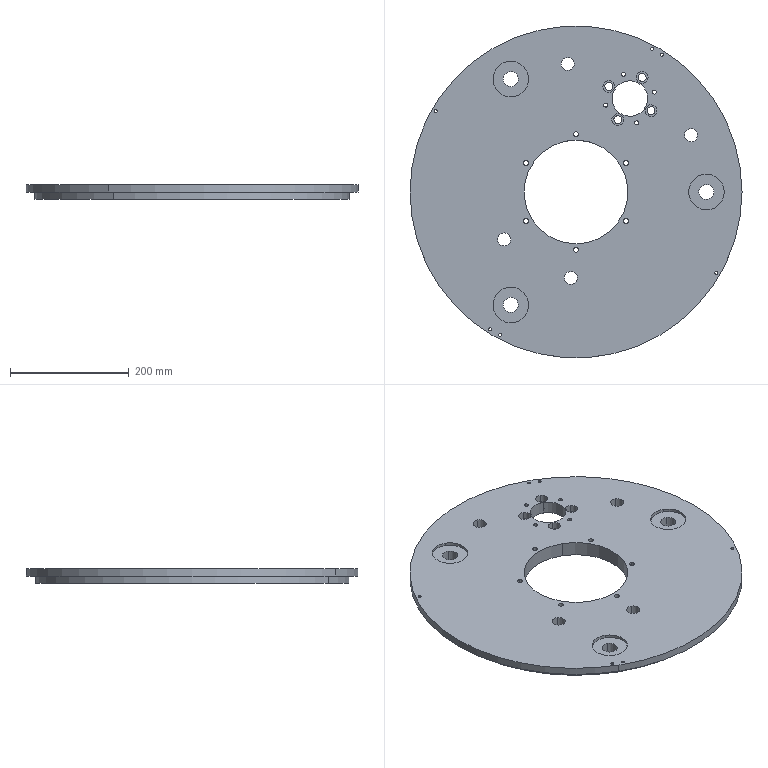Component | SolidWorks | KLHFH002Turntable-1 | 1 solid | 89 faces | box 560 x 560 x 25 mm | volume 4987410 mm3 | cylinder 78 | plane 11 | commonest cylinder face diameters 8.5 x12 5 x12 22 x8 60 x8 20 x8 6.8 x8 13.5 x8 25.5 x6 | material Plain Carbon Steel
build123d program:
from build123d import *

# Parameters (mm, degrees)
SKETCH1_R                                          = 265
BOSS_EXTRUDE1_DEPTH                                = 12.5
SKETCH2_R                                          = 30
SKETCH2_R_2                                        = 35
CUT_EXTRUDE1_DEPTH                                 = 376.6
HOLE_SIZE_ACCORDING_TO_TYPE_1_OF_HEXAG_D           = 13.5
HOLE_SIZE_ACCORDING_TO_TYPE_1_OF_HEXAG_DEPTH       = 38.75
HOLE_SIZE_ACCORDING_TO_TYPE_1_OF_HEXAG_CBORE_D     = 20
HOLE_SIZE_ACCORDING_TO_TYPE_1_OF_HEXAG_CBORE_DEPTH = 13
HOLE_SIZE_ACCORDING_TO_TYPE_1_OF_HEXAG_TIP         = 4.056
M8_TAPPED_HOLE1_D                                  = 6.8
SKETCH7_R                                          = 65
CUT_EXTRUDE2_DEPTH                                 = 3
HOLE_SIZE_ACCORDING_TO_TYPE_2_OF_HEXAG_D           = 9
HOLE_SIZE_ACCORDING_TO_TYPE_2_OF_HEXAG_CBORE_D     = 15
HOLE_SIZE_ACCORDING_TO_TYPE_2_OF_HEXAG_CBORE_DEPTH = 9
SKETCH10_R                                         = 8
CUT_EXTRUDE3_DEPTH                                 = 3
M6_TAPPED_HOLE2_D                                  = 5
SKETCH15_R                                         = 30
CUT_EXTRUDE4_DEPTH                                 = 5
F_25_5_25_5_DIAMETER_HOLE1_D                       = 25.5
CIRPATTERN1_COUNT                                  = 3
M10_TAPPED_HOLE1_D                                 = 8.5
SKETCH20_R                                         = 11
CUT_EXTRUDE5_DEPTH                                 = 376.6
SKETCH21_R                                         = 11
CUT_EXTRUDE6_DEPTH                                 = 376.6
BOSS_EXTRUDE2_START                                = -12.5
SKETCH22_R                                         = 280
SKETCH22_R_2                                       = 265
BOSS_EXTRUDE2_DEPTH                                = 12.5
M6_TAPPED_HOLE3_D                                  = 5
SKETCH25_R                                         = 87.5
CUT_EXTRUDE7_DEPTH                                 = 397.768
M10_TAPPED_HOLE2_D                                 = 8.5
CIRPATTERN2_COUNT                                  = 6


with BuildPart() as part:
    # Sketch1 → Boss-Extrude1 (new, symmetric)
    with BuildSketch(Plane.XY):
        Circle(SKETCH1_R)
    extrude(amount=BOSS_EXTRUDE1_DEPTH, both=True)

    # Sketch2 → Cut-Extrude1 (cut, through all)
    with BuildSketch(Plane.XY.offset(12.5)):
        with Locations((-182, 0)):
            Circle(SKETCH2_R)
        Circle(SKETCH2_R_2)
    extrude(amount=-CUT_EXTRUDE1_DEPTH, mode=Mode.SUBTRACT)

    # Hole Size _according to_ Type 1 of Hexag
    with Locations(Plane(origin=(0, 0, -12.5), x_dir=(-1, 0, 0), z_dir=(0, 0, -1))):
        with Locations((141, 0), (182, 41), (223, 0), (182, -41)):
            CounterBoreHole(HOLE_SIZE_ACCORDING_TO_TYPE_1_OF_HEXAG_D / 2, HOLE_SIZE_ACCORDING_TO_TYPE_1_OF_HEXAG_CBORE_D / 2, HOLE_SIZE_ACCORDING_TO_TYPE_1_OF_HEXAG_CBORE_DEPTH, depth=HOLE_SIZE_ACCORDING_TO_TYPE_1_OF_HEXAG_DEPTH)
            with Locations((0, 0, -(HOLE_SIZE_ACCORDING_TO_TYPE_1_OF_HEXAG_DEPTH + HOLE_SIZE_ACCORDING_TO_TYPE_1_OF_HEXAG_TIP / 2))):  # 118° drill point
                Cone(0, HOLE_SIZE_ACCORDING_TO_TYPE_1_OF_HEXAG_D / 2, HOLE_SIZE_ACCORDING_TO_TYPE_1_OF_HEXAG_TIP, mode=Mode.SUBTRACT)

    # M8 Tapped Hole1 (through all)
    with Locations(Plane(origin=(0, 0, -12.5), x_dir=(-1, 0, 0), z_dir=(0, 0, -1))):
        with Locations((212, 30), (212, -30), (152, -30), (152, 30)):
            Hole(M8_TAPPED_HOLE1_D / 2)

    # Sketch7 → Cut-Extrude2 (cut)
    with BuildSketch(Plane.XY.offset(12.5)):
        with Locations((-182, 0)):
            Circle(SKETCH7_R)
    extrude(amount=-CUT_EXTRUDE2_DEPTH, mode=Mode.SUBTRACT)

    # Hole Size _according to_ Type 2 of Hexag (through all)
    with Locations(Plane(origin=(0, 0, -12.5), x_dir=(1, 0, 0), z_dir=(0, 0, -1))):
        with Locations((-50, 0), (50, 0)):
            CounterBoreHole(HOLE_SIZE_ACCORDING_TO_TYPE_2_OF_HEXAG_D / 2, HOLE_SIZE_ACCORDING_TO_TYPE_2_OF_HEXAG_CBORE_D / 2, HOLE_SIZE_ACCORDING_TO_TYPE_2_OF_HEXAG_CBORE_DEPTH)

    # Sketch10 → Cut-Extrude3 (cut)
    with BuildSketch(Plane.XY.offset(12.5)):
        with Locations((-50, 0)):
            Circle(SKETCH10_R)
        with Locations((50, 0)):
            Circle(SKETCH10_R)
    extrude(amount=-CUT_EXTRUDE3_DEPTH, mode=Mode.SUBTRACT)

    # M6 Tapped Hole2 (through all)
    with Locations(Plane.XY.offset(12.5)):
        with Locations((-60, -40), (-77.5, -20), (-77.5, 20), (-60, 40), (-10, 40), (10, 40), (-10, -40), (10, -40), (60, -40), (77.5, -20), (77.5, 20), (60, 40)):
            Hole(M6_TAPPED_HOLE2_D / 2)

    # Sketch15 → Cut-Extrude4 (cut)
    with BuildSketch(Plane(origin=(0, 0, -12.5), x_dir=(-1, 0, 0), z_dir=(0, 0, -1))):
        with Locations((-220, 0)):
            Circle(SKETCH15_R)
    cut_extrude4 = extrude(amount=-CUT_EXTRUDE4_DEPTH, mode=Mode.SUBTRACT)

    # 25.5 _25.5_ Diameter Hole1 (through all)
    with Locations(Plane.XY.offset(12.5)):
        with Locations((220, 0)):
            f_25_5_25_5_diameter_hole1 = Hole(F_25_5_25_5_DIAMETER_HOLE1_D / 2)

    # CirPattern1: Cut-Extrude4, 25.5 _25.5_ Diameter Hole1 ×3 about axis
    cirpattern1_axis = Axis((0, 0, 0), (0, 0, 1))
    add([cut_extrude4.rotate(cirpattern1_axis, i * 360 / CIRPATTERN1_COUNT) for i in range(1, CIRPATTERN1_COUNT)], mode=Mode.SUBTRACT)
    add([f_25_5_25_5_diameter_hole1.rotate(cirpattern1_axis, i * 360 / CIRPATTERN1_COUNT) for i in range(1, CIRPATTERN1_COUNT)], mode=Mode.SUBTRACT)

    # M10 Tapped Hole1 (through all)
    with Locations(Plane(origin=(0, 0, -12.5), x_dir=(-1, 0, 0), z_dir=(0, 0, -1))):
        with Locations((-47, 47), (47, 47), (-47, -47), (47, -47)):
            Hole(M10_TAPPED_HOLE1_D / 2)

    # Sketch20 → Cut-Extrude5 (cut, through all)
    with BuildSketch(Plane.XY.offset(12.5)):
        with Locations((130, 65)):
            Circle(SKETCH20_R)
        with Locations((130, -65)):
            Circle(SKETCH20_R)
    extrude(amount=-CUT_EXTRUDE5_DEPTH, mode=Mode.SUBTRACT)

    # Sketch21 → Cut-Extrude6 (cut, through all)
    with BuildSketch(Plane.XY.offset(12.5)):
        with Locations((-180, -120)):
            Circle(SKETCH21_R)
        with Locations((-180, 120)):
            Circle(SKETCH21_R)
    extrude(amount=-CUT_EXTRUDE6_DEPTH, mode=Mode.SUBTRACT)

    # Sketch22 → Boss-Extrude2 (add)
    with BuildSketch(Plane(origin=(0, 0, -12.5), x_dir=(-1, 0, 0), z_dir=(0, 0, -1)).offset(BOSS_EXTRUDE2_START)):
        Circle(SKETCH22_R)
        Circle(SKETCH22_R_2, mode=Mode.SUBTRACT)
    extrude(amount=BOSS_EXTRUDE2_DEPTH)

    # M6 Tapped Hole3 (through all)
    with Locations(Plane.XY):
        with Locations((0, -273), (272.834, -9.528), (272.834, 9.528), (-272.834, -9.528), (-273, 9.533), (0, 273)):
            Hole(M6_TAPPED_HOLE3_D / 2)

    # Sketch25 → Cut-Extrude7 (cut, through all)
    with BuildSketch(Plane.XY.offset(12.5)):
        Circle(SKETCH25_R)
    extrude(amount=-CUT_EXTRUDE7_DEPTH, mode=Mode.SUBTRACT)

    # M10 Tapped Hole2 (through all)
    with Locations(Plane.XY.offset(12.5)):
        with Locations((0, -97.5)):
            m10_tapped_hole2 = Hole(M10_TAPPED_HOLE2_D / 2)

    # CirPattern2: M10 Tapped Hole2 ×6 about axis
    cirpattern2_axis = Axis((0, 0, 0), (0, 0, 1))
    for i in range(1, CIRPATTERN2_COUNT):
        add(m10_tapped_hole2.rotate(cirpattern2_axis, i * 360 / CIRPATTERN2_COUNT), mode=Mode.SUBTRACT)


solid = part.part

# Placed as in the assembly
solid = solid.moved(Location((0, 0, -165), (-180, 0, 120)))